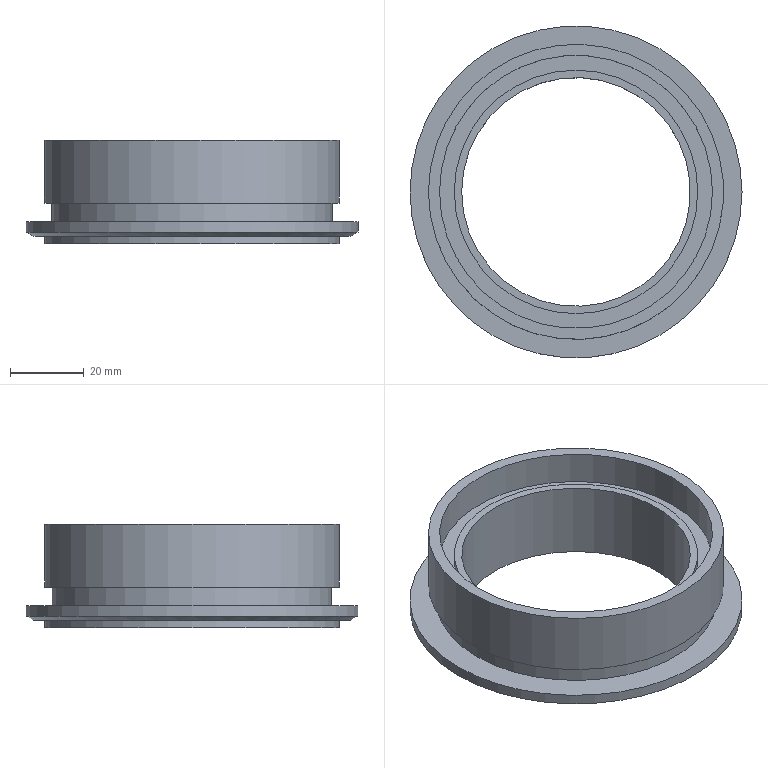Component | NX | CH3404_19_3-2 | 1 solid | 15 faces | box 90 x 90 x 28 mm | volume 48046 mm3 | cylinder 7 | plane 7 | cone 1 | commonest cylinder face diameters 80 x2 90 x1 62 x1 66 x1 74 x1 76 x1
STEP:
#1=CARTESIAN_POINT('',(0.,0.,0.));
#2=DIRECTION('',(0.,0.,1.));
#3=DIRECTION('',(1.,0.,0.));
#4=AXIS2_PLACEMENT_3D('',#1,#2,#3);
#5=CARTESIAN_POINT('',(45.,0.,77.155));
#6=VERTEX_POINT('',#5);
#7=CARTESIAN_POINT('',(-45.,0.,77.155));
#8=VERTEX_POINT('',#7);
#9=CARTESIAN_POINT('',(0.,0.,77.155));
#10=DIRECTION('',(0.,0.,1.));
#11=DIRECTION('',(1.,0.,0.));
#12=AXIS2_PLACEMENT_3D('',#9,#10,#11);
#13=CIRCLE('',#12,45.);
#14=CARTESIAN_POINT('',(0.,0.,74.));
#15=DIRECTION('',(0.,0.,-1.));
#16=DIRECTION('',(-1.,0.,0.));
#17=AXIS2_PLACEMENT_3D('',#14,#15,#16);
#18=CYLINDRICAL_SURFACE('',#17,45.);
#19=CARTESIAN_POINT('',(3.142,-3.155));
#20=DIRECTION('',(-1.,0.));
#21=VECTOR('',#20,1.);
#22=LINE('',#19,#21);
#23=(GEOMETRIC_REPRESENTATION_CONTEXT(2)PARAMETRIC_REPRESENTATION_CONTEXT()REPRESENTATION_CONTEXT('',''));
#24=DEFINITIONAL_REPRESENTATION('',(#22),#23);
#25=PCURVE('',#18,#24);
#26=CARTESIAN_POINT('',(0.,0.,76.));
#27=DIRECTION('',(0.,0.,1.));
#28=DIRECTION('',(1.,0.,0.));
#29=AXIS2_PLACEMENT_3D('',#26,#27,#28);
#30=CONICAL_SURFACE('',#29,43.,1.047);
#31=CARTESIAN_POINT('',(0.,1.155));
#32=DIRECTION('',(1.,0.));
#33=VECTOR('',#32,1.);
#34=LINE('',#31,#33);
#35=(GEOMETRIC_REPRESENTATION_CONTEXT(2)PARAMETRIC_REPRESENTATION_CONTEXT()REPRESENTATION_CONTEXT('',''));
#36=DEFINITIONAL_REPRESENTATION('',(#34),#35);
#37=PCURVE('',#30,#36);
#38=SURFACE_CURVE('',#13,(#25,#37),.PCURVE_S1.);
#39=EDGE_CURVE('',#6,#8,#38,.T.);
#40=ORIENTED_EDGE('',*,*,#39,.T.);
#41=CARTESIAN_POINT('',(-45.,0.,80.));
#42=VERTEX_POINT('',#41);
#43=CARTESIAN_POINT('',(-45.,-0.,80.));
#44=CARTESIAN_POINT('',(-45.,-0.,77.155));
#45=B_SPLINE_CURVE_WITH_KNOTS('',1,(#43,#44),.UNSPECIFIED.,.F.,.F.,(2,2),(-6.,-3.155),.PIECEWISE_BEZIER_KNOTS.);
#46=CARTESIAN_POINT('',(0.,0.));
#47=DIRECTION('',(0.,1.));
#48=VECTOR('',#47,1.);
#49=LINE('',#46,#48);
#50=(GEOMETRIC_REPRESENTATION_CONTEXT(2)PARAMETRIC_REPRESENTATION_CONTEXT()REPRESENTATION_CONTEXT('',''));
#51=DEFINITIONAL_REPRESENTATION('',(#49),#50);
#52=PCURVE('',#18,#51);
#53=CARTESIAN_POINT('',(6.283,0.));
#54=DIRECTION('',(0.,1.));
#55=VECTOR('',#54,1.);
#56=LINE('',#53,#55);
#57=(GEOMETRIC_REPRESENTATION_CONTEXT(2)PARAMETRIC_REPRESENTATION_CONTEXT()REPRESENTATION_CONTEXT('',''));
#58=DEFINITIONAL_REPRESENTATION('',(#56),#57);
#59=PCURVE('',#18,#58);
#60=SEAM_CURVE('',#45,(#52,#59),.PCURVE_S1.);
#61=EDGE_CURVE('',#42,#8,#60,.T.);
#62=ORIENTED_EDGE('',*,*,#61,.F.);
#63=CARTESIAN_POINT('',(0.,0.,80.));
#64=DIRECTION('',(0.,0.,-1.));
#65=DIRECTION('',(-1.,0.,0.));
#66=AXIS2_PLACEMENT_3D('',#63,#64,#65);
#67=CIRCLE('',#66,45.);
#68=CARTESIAN_POINT('',(0.,-6.));
#69=DIRECTION('',(1.,0.));
#70=VECTOR('',#69,1.);
#71=LINE('',#68,#70);
#72=(GEOMETRIC_REPRESENTATION_CONTEXT(2)PARAMETRIC_REPRESENTATION_CONTEXT()REPRESENTATION_CONTEXT('',''));
#73=DEFINITIONAL_REPRESENTATION('',(#71),#72);
#74=PCURVE('',#18,#73);
#75=CARTESIAN_POINT('',(0.,-38.,80.));
#76=DIRECTION('',(0.,0.,-1.));
#77=DIRECTION('',(-1.,0.,0.));
#78=AXIS2_PLACEMENT_3D('',#75,#76,#77);
#79=PLANE('',#78);
#80=CARTESIAN_POINT('',(0.,38.));
#81=DIRECTION('',(1.,0.));
#82=AXIS2_PLACEMENT_2D('',#80,#81);
#83=CIRCLE('',#82,45.);
#84=(GEOMETRIC_REPRESENTATION_CONTEXT(2)PARAMETRIC_REPRESENTATION_CONTEXT()REPRESENTATION_CONTEXT('',''));
#85=DEFINITIONAL_REPRESENTATION('',(#83),#84);
#86=PCURVE('',#79,#85);
#87=SURFACE_CURVE('',#67,(#74,#86),.PCURVE_S1.);
#88=EDGE_CURVE('',#42,#42,#87,.T.);
#89=ORIENTED_EDGE('',*,*,#88,.T.);
#90=ORIENTED_EDGE('',*,*,#61,.T.);
#91=CARTESIAN_POINT('',(0.,0.,77.155));
#92=DIRECTION('',(0.,0.,1.));
#93=DIRECTION('',(1.,0.,0.));
#94=AXIS2_PLACEMENT_3D('',#91,#92,#93);
#95=CIRCLE('',#94,45.);
#96=CARTESIAN_POINT('',(9.425,-3.155));
#97=DIRECTION('',(-1.,0.));
#98=VECTOR('',#97,1.);
#99=LINE('',#96,#98);
#100=(GEOMETRIC_REPRESENTATION_CONTEXT(2)PARAMETRIC_REPRESENTATION_CONTEXT()REPRESENTATION_CONTEXT('',''));
#101=DEFINITIONAL_REPRESENTATION('',(#99),#100);
#102=PCURVE('',#18,#101);
#103=CARTESIAN_POINT('',(0.,1.155));
#104=DIRECTION('',(1.,0.));
#105=VECTOR('',#104,1.);
#106=LINE('',#103,#105);
#107=(GEOMETRIC_REPRESENTATION_CONTEXT(2)PARAMETRIC_REPRESENTATION_CONTEXT()REPRESENTATION_CONTEXT('',''));
#108=DEFINITIONAL_REPRESENTATION('',(#106),#107);
#109=PCURVE('',#30,#108);
#110=SURFACE_CURVE('',#95,(#102,#109),.PCURVE_S1.);
#111=EDGE_CURVE('',#8,#6,#110,.T.);
#112=ORIENTED_EDGE('',*,*,#111,.T.);
#113=EDGE_LOOP('',(#40,#62,#89,#90,#112));
#114=FACE_BOUND('',#113,.T.);
#115=ADVANCED_FACE('',(#114),#18,.T.);
#116=CARTESIAN_POINT('',(43.,0.,76.));
#117=VERTEX_POINT('',#116);
#118=CARTESIAN_POINT('',(0.,0.,76.));
#119=DIRECTION('',(0.,0.,-1.));
#120=DIRECTION('',(1.,0.,0.));
#121=AXIS2_PLACEMENT_3D('',#118,#119,#120);
#122=CIRCLE('',#121,43.);
#123=CARTESIAN_POINT('',(0.,-45.,76.));
#124=DIRECTION('',(0.,0.,1.));
#125=DIRECTION('',(1.,0.,0.));
#126=AXIS2_PLACEMENT_3D('',#123,#124,#125);
#127=PLANE('',#126);
#128=CARTESIAN_POINT('',(43.,45.));
#129=CARTESIAN_POINT('',(43.,-29.478));
#130=CARTESIAN_POINT('',(-21.5,7.761));
#131=CARTESIAN_POINT('',(-86.,45.));
#132=CARTESIAN_POINT('',(-21.5,82.239));
#133=CARTESIAN_POINT('',(43.,119.478));
#134=CARTESIAN_POINT('',(43.,45.));
#135=(BOUNDED_CURVE()B_SPLINE_CURVE(2,(#128,#129,#130,#131,#132,#133,#134),.UNSPECIFIED.,.T.,.F.)B_SPLINE_CURVE_WITH_KNOTS((1,2,2,2,2,1),(-2.094,0.,2.094,4.189,6.283,8.378),.UNSPECIFIED.)CURVE()GEOMETRIC_REPRESENTATION_ITEM()RATIONAL_B_SPLINE_CURVE((1.,0.5,1.,0.5,1.,0.5,1.))REPRESENTATION_ITEM(''));
#136=(GEOMETRIC_REPRESENTATION_CONTEXT(2)PARAMETRIC_REPRESENTATION_CONTEXT()REPRESENTATION_CONTEXT('',''));
#137=DEFINITIONAL_REPRESENTATION('',(#135),#136);
#138=PCURVE('',#127,#137);
#139=CARTESIAN_POINT('',(6.283,0.));
#140=DIRECTION('',(-1.,0.));
#141=VECTOR('',#140,1.);
#142=LINE('',#139,#141);
#143=(GEOMETRIC_REPRESENTATION_CONTEXT(2)PARAMETRIC_REPRESENTATION_CONTEXT()REPRESENTATION_CONTEXT('',''));
#144=DEFINITIONAL_REPRESENTATION('',(#142),#143);
#145=PCURVE('',#30,#144);
#146=SURFACE_CURVE('',#122,(#138,#145),.PCURVE_S1.);
#147=EDGE_CURVE('',#117,#117,#146,.T.);
#148=ORIENTED_EDGE('',*,*,#147,.T.);
#149=EDGE_LOOP('',(#148));
#150=FACE_BOUND('',#149,.T.);
#151=CARTESIAN_POINT('',(-40.,0.,76.));
#152=VERTEX_POINT('',#151);
#153=CARTESIAN_POINT('',(0.,0.,76.));
#154=DIRECTION('',(0.,0.,-1.));
#155=DIRECTION('',(-1.,0.,0.));
#156=AXIS2_PLACEMENT_3D('',#153,#154,#155);
#157=CIRCLE('',#156,40.);
#158=CARTESIAN_POINT('',(-40.,45.));
#159=CARTESIAN_POINT('',(-40.,114.282));
#160=CARTESIAN_POINT('',(20.,79.641));
#161=CARTESIAN_POINT('',(80.,45.));
#162=CARTESIAN_POINT('',(20.,10.359));
#163=CARTESIAN_POINT('',(-40.,-24.282));
#164=CARTESIAN_POINT('',(-40.,45.));
#165=(BOUNDED_CURVE()B_SPLINE_CURVE(2,(#158,#159,#160,#161,#162,#163,#164),.UNSPECIFIED.,.T.,.F.)B_SPLINE_CURVE_WITH_KNOTS((1,2,2,2,2,1),(-2.094,0.,2.094,4.189,6.283,8.378),.UNSPECIFIED.)CURVE()GEOMETRIC_REPRESENTATION_ITEM()RATIONAL_B_SPLINE_CURVE((1.,0.5,1.,0.5,1.,0.5,1.))REPRESENTATION_ITEM(''));
#166=(GEOMETRIC_REPRESENTATION_CONTEXT(2)PARAMETRIC_REPRESENTATION_CONTEXT()REPRESENTATION_CONTEXT('',''));
#167=DEFINITIONAL_REPRESENTATION('',(#165),#166);
#168=PCURVE('',#127,#167);
#169=CARTESIAN_POINT('',(0.,0.,74.));
#170=DIRECTION('',(0.,0.,-1.));
#171=DIRECTION('',(-1.,0.,0.));
#172=AXIS2_PLACEMENT_3D('',#169,#170,#171);
#173=CYLINDRICAL_SURFACE('',#172,40.);
#174=CARTESIAN_POINT('',(0.,-2.));
#175=DIRECTION('',(1.,0.));
#176=VECTOR('',#175,1.);
#177=LINE('',#174,#176);
#178=(GEOMETRIC_REPRESENTATION_CONTEXT(2)PARAMETRIC_REPRESENTATION_CONTEXT()REPRESENTATION_CONTEXT('',''));
#179=DEFINITIONAL_REPRESENTATION('',(#177),#178);
#180=PCURVE('',#173,#179);
#181=SURFACE_CURVE('',#157,(#168,#180),.PCURVE_S1.);
#182=EDGE_CURVE('',#152,#152,#181,.T.);
#183=ORIENTED_EDGE('',*,*,#182,.F.);
#184=EDGE_LOOP('',(#183));
#185=FACE_BOUND('',#184,.T.);
#186=ADVANCED_FACE('',(#150,#185),#127,.F.);
#187=CARTESIAN_POINT('',(-40.,0.,74.));
#188=VERTEX_POINT('',#187);
#189=CARTESIAN_POINT('',(0.,0.,74.));
#190=DIRECTION('',(0.,0.,-1.));
#191=DIRECTION('',(-1.,0.,0.));
#192=AXIS2_PLACEMENT_3D('',#189,#190,#191);
#193=CIRCLE('',#192,40.);
#194=CARTESIAN_POINT('',(0.,0.));
#195=DIRECTION('',(1.,0.));
#196=VECTOR('',#195,1.);
#197=LINE('',#194,#196);
#198=(GEOMETRIC_REPRESENTATION_CONTEXT(2)PARAMETRIC_REPRESENTATION_CONTEXT()REPRESENTATION_CONTEXT('',''));
#199=DEFINITIONAL_REPRESENTATION('',(#197),#198);
#200=PCURVE('',#173,#199);
#201=CARTESIAN_POINT('',(0.,-40.,74.));
#202=DIRECTION('',(0.,0.,1.));
#203=DIRECTION('',(1.,0.,0.));
#204=AXIS2_PLACEMENT_3D('',#201,#202,#203);
#205=PLANE('',#204);
#206=CARTESIAN_POINT('',(-40.,40.));
#207=CARTESIAN_POINT('',(-40.,109.282));
#208=CARTESIAN_POINT('',(20.,74.641));
#209=CARTESIAN_POINT('',(80.,40.));
#210=CARTESIAN_POINT('',(20.,5.359));
#211=CARTESIAN_POINT('',(-40.,-29.282));
#212=CARTESIAN_POINT('',(-40.,40.));
#213=(BOUNDED_CURVE()B_SPLINE_CURVE(2,(#206,#207,#208,#209,#210,#211,#212),.UNSPECIFIED.,.T.,.F.)B_SPLINE_CURVE_WITH_KNOTS((1,2,2,2,2,1),(-2.094,0.,2.094,4.189,6.283,8.378),.UNSPECIFIED.)CURVE()GEOMETRIC_REPRESENTATION_ITEM()RATIONAL_B_SPLINE_CURVE((1.,0.5,1.,0.5,1.,0.5,1.))REPRESENTATION_ITEM(''));
#214=(GEOMETRIC_REPRESENTATION_CONTEXT(2)PARAMETRIC_REPRESENTATION_CONTEXT()REPRESENTATION_CONTEXT('',''));
#215=DEFINITIONAL_REPRESENTATION('',(#213),#214);
#216=PCURVE('',#205,#215);
#217=SURFACE_CURVE('',#193,(#200,#216),.PCURVE_S1.);
#218=EDGE_CURVE('',#188,#188,#217,.T.);
#219=ORIENTED_EDGE('',*,*,#218,.F.);
#220=CARTESIAN_POINT('',(-40.,-0.,76.));
#221=CARTESIAN_POINT('',(-40.,-0.,74.));
#222=B_SPLINE_CURVE_WITH_KNOTS('',1,(#220,#221),.UNSPECIFIED.,.F.,.F.,(2,2),(-2.,0.),.PIECEWISE_BEZIER_KNOTS.);
#223=CARTESIAN_POINT('',(0.,0.));
#224=DIRECTION('',(0.,1.));
#225=VECTOR('',#224,1.);
#226=LINE('',#223,#225);
#227=(GEOMETRIC_REPRESENTATION_CONTEXT(2)PARAMETRIC_REPRESENTATION_CONTEXT()REPRESENTATION_CONTEXT('',''));
#228=DEFINITIONAL_REPRESENTATION('',(#226),#227);
#229=PCURVE('',#173,#228);
#230=CARTESIAN_POINT('',(6.283,0.));
#231=DIRECTION('',(0.,1.));
#232=VECTOR('',#231,1.);
#233=LINE('',#230,#232);
#234=(GEOMETRIC_REPRESENTATION_CONTEXT(2)PARAMETRIC_REPRESENTATION_CONTEXT()REPRESENTATION_CONTEXT('',''));
#235=DEFINITIONAL_REPRESENTATION('',(#233),#234);
#236=PCURVE('',#173,#235);
#237=SEAM_CURVE('',#222,(#229,#236),.PCURVE_S1.);
#238=EDGE_CURVE('',#152,#188,#237,.T.);
#239=ORIENTED_EDGE('',*,*,#238,.F.);
#240=ORIENTED_EDGE('',*,*,#182,.T.);
#241=ORIENTED_EDGE('',*,*,#238,.T.);
#242=EDGE_LOOP('',(#219,#239,#240,#241));
#243=FACE_BOUND('',#242,.T.);
#244=ADVANCED_FACE('',(#243),#173,.T.);
#245=CARTESIAN_POINT('',(-31.,0.,74.));
#246=VERTEX_POINT('',#245);
#247=CARTESIAN_POINT('',(0.,0.,74.));
#248=DIRECTION('',(0.,0.,-1.));
#249=DIRECTION('',(-1.,0.,0.));
#250=AXIS2_PLACEMENT_3D('',#247,#248,#249);
#251=CIRCLE('',#250,31.);
#252=CARTESIAN_POINT('',(-31.,40.));
#253=CARTESIAN_POINT('',(-31.,93.694));
#254=CARTESIAN_POINT('',(15.5,66.847));
#255=CARTESIAN_POINT('',(62.,40.));
#256=CARTESIAN_POINT('',(15.5,13.153));
#257=CARTESIAN_POINT('',(-31.,-13.694));
#258=CARTESIAN_POINT('',(-31.,40.));
#259=(BOUNDED_CURVE()B_SPLINE_CURVE(2,(#252,#253,#254,#255,#256,#257,#258),.UNSPECIFIED.,.T.,.F.)B_SPLINE_CURVE_WITH_KNOTS((1,2,2,2,2,1),(-2.094,0.,2.094,4.189,6.283,8.378),.UNSPECIFIED.)CURVE()GEOMETRIC_REPRESENTATION_ITEM()RATIONAL_B_SPLINE_CURVE((1.,0.5,1.,0.5,1.,0.5,1.))REPRESENTATION_ITEM(''));
#260=(GEOMETRIC_REPRESENTATION_CONTEXT(2)PARAMETRIC_REPRESENTATION_CONTEXT()REPRESENTATION_CONTEXT('',''));
#261=DEFINITIONAL_REPRESENTATION('',(#259),#260);
#262=PCURVE('',#205,#261);
#263=CARTESIAN_POINT('',(0.,0.,74.));
#264=DIRECTION('',(0.,0.,-1.));
#265=DIRECTION('',(-1.,0.,0.));
#266=AXIS2_PLACEMENT_3D('',#263,#264,#265);
#267=CYLINDRICAL_SURFACE('',#266,31.);
#268=CARTESIAN_POINT('',(0.,0.));
#269=DIRECTION('',(1.,0.));
#270=VECTOR('',#269,1.);
#271=LINE('',#268,#270);
#272=(GEOMETRIC_REPRESENTATION_CONTEXT(2)PARAMETRIC_REPRESENTATION_CONTEXT()REPRESENTATION_CONTEXT('',''));
#273=DEFINITIONAL_REPRESENTATION('',(#271),#272);
#274=PCURVE('',#267,#273);
#275=SURFACE_CURVE('',#251,(#262,#274),.PCURVE_S1.);
#276=EDGE_CURVE('',#246,#246,#275,.T.);
#277=ORIENTED_EDGE('',*,*,#276,.F.);
#278=EDGE_LOOP('',(#277));
#279=FACE_BOUND('',#278,.T.);
#280=ORIENTED_EDGE('',*,*,#218,.T.);
#281=EDGE_LOOP('',(#280));
#282=FACE_BOUND('',#281,.T.);
#283=ADVANCED_FACE('',(#279,#282),#205,.F.);
#284=CARTESIAN_POINT('',(-31.,0.,95.));
#285=VERTEX_POINT('',#284);
#286=CARTESIAN_POINT('',(0.,0.,95.));
#287=DIRECTION('',(0.,0.,-1.));
#288=DIRECTION('',(-1.,0.,0.));
#289=AXIS2_PLACEMENT_3D('',#286,#287,#288);
#290=CIRCLE('',#289,31.);
#291=CARTESIAN_POINT('',(0.,-21.));
#292=DIRECTION('',(1.,0.));
#293=VECTOR('',#292,1.);
#294=LINE('',#291,#293);
#295=(GEOMETRIC_REPRESENTATION_CONTEXT(2)PARAMETRIC_REPRESENTATION_CONTEXT()REPRESENTATION_CONTEXT('',''));
#296=DEFINITIONAL_REPRESENTATION('',(#294),#295);
#297=PCURVE('',#267,#296);
#298=CARTESIAN_POINT('',(0.,-31.,95.));
#299=DIRECTION('',(0.,0.,-1.));
#300=DIRECTION('',(-1.,0.,0.));
#301=AXIS2_PLACEMENT_3D('',#298,#299,#300);
#302=PLANE('',#301);
#303=CARTESIAN_POINT('',(0.,31.));
#304=DIRECTION('',(1.,0.));
#305=AXIS2_PLACEMENT_2D('',#303,#304);
#306=CIRCLE('',#305,31.);
#307=(GEOMETRIC_REPRESENTATION_CONTEXT(2)PARAMETRIC_REPRESENTATION_CONTEXT()REPRESENTATION_CONTEXT('',''));
#308=DEFINITIONAL_REPRESENTATION('',(#306),#307);
#309=PCURVE('',#302,#308);
#310=SURFACE_CURVE('',#290,(#297,#309),.PCURVE_S1.);
#311=EDGE_CURVE('',#285,#285,#310,.T.);
#312=ORIENTED_EDGE('',*,*,#311,.T.);
#313=CARTESIAN_POINT('',(-31.,0.,95.));
#314=CARTESIAN_POINT('',(-31.,0.,74.));
#315=B_SPLINE_CURVE_WITH_KNOTS('',1,(#313,#314),.UNSPECIFIED.,.F.,.F.,(2,2),(-21.,0.),.PIECEWISE_BEZIER_KNOTS.);
#316=CARTESIAN_POINT('',(6.283,0.));
#317=DIRECTION('',(0.,1.));
#318=VECTOR('',#317,1.);
#319=LINE('',#316,#318);
#320=(GEOMETRIC_REPRESENTATION_CONTEXT(2)PARAMETRIC_REPRESENTATION_CONTEXT()REPRESENTATION_CONTEXT('',''));
#321=DEFINITIONAL_REPRESENTATION('',(#319),#320);
#322=PCURVE('',#267,#321);
#323=CARTESIAN_POINT('',(0.,0.));
#324=DIRECTION('',(0.,1.));
#325=VECTOR('',#324,1.);
#326=LINE('',#323,#325);
#327=(GEOMETRIC_REPRESENTATION_CONTEXT(2)PARAMETRIC_REPRESENTATION_CONTEXT()REPRESENTATION_CONTEXT('',''));
#328=DEFINITIONAL_REPRESENTATION('',(#326),#327);
#329=PCURVE('',#267,#328);
#330=SEAM_CURVE('',#315,(#322,#329),.PCURVE_S1.);
#331=EDGE_CURVE('',#285,#246,#330,.T.);
#332=ORIENTED_EDGE('',*,*,#331,.T.);
#333=ORIENTED_EDGE('',*,*,#276,.F.);
#334=ORIENTED_EDGE('',*,*,#331,.F.);
#335=EDGE_LOOP('',(#312,#332,#333,#334));
#336=FACE_BOUND('',#335,.F.);
#337=ADVANCED_FACE('',(#336),#267,.F.);
#338=CARTESIAN_POINT('',(-33.,0.,95.));
#339=VERTEX_POINT('',#338);
#340=CARTESIAN_POINT('',(0.,0.,95.));
#341=DIRECTION('',(0.,0.,-1.));
#342=DIRECTION('',(-1.,0.,0.));
#343=AXIS2_PLACEMENT_3D('',#340,#341,#342);
#344=CIRCLE('',#343,33.);
#345=CARTESIAN_POINT('',(0.,31.));
#346=DIRECTION('',(1.,0.));
#347=AXIS2_PLACEMENT_2D('',#345,#346);
#348=CIRCLE('',#347,33.);
#349=(GEOMETRIC_REPRESENTATION_CONTEXT(2)PARAMETRIC_REPRESENTATION_CONTEXT()REPRESENTATION_CONTEXT('',''));
#350=DEFINITIONAL_REPRESENTATION('',(#348),#349);
#351=PCURVE('',#302,#350);
#352=CARTESIAN_POINT('',(0.,0.,74.));
#353=DIRECTION('',(0.,0.,-1.));
#354=DIRECTION('',(-1.,0.,0.));
#355=AXIS2_PLACEMENT_3D('',#352,#353,#354);
#356=CYLINDRICAL_SURFACE('',#355,33.);
#357=CARTESIAN_POINT('',(0.,-21.));
#358=DIRECTION('',(1.,0.));
#359=VECTOR('',#358,1.);
#360=LINE('',#357,#359);
#361=(GEOMETRIC_REPRESENTATION_CONTEXT(2)PARAMETRIC_REPRESENTATION_CONTEXT()REPRESENTATION_CONTEXT('',''));
#362=DEFINITIONAL_REPRESENTATION('',(#360),#361);
#363=PCURVE('',#356,#362);
#364=SURFACE_CURVE('',#344,(#351,#363),.PCURVE_S1.);
#365=EDGE_CURVE('',#339,#339,#364,.T.);
#366=ORIENTED_EDGE('',*,*,#365,.F.);
#367=EDGE_LOOP('',(#366));
#368=FACE_BOUND('',#367,.T.);
#369=ORIENTED_EDGE('',*,*,#311,.T.);
#370=EDGE_LOOP('',(#369));
#371=FACE_BOUND('',#370,.T.);
#372=ADVANCED_FACE('',(#368,#371),#302,.F.);
#373=CARTESIAN_POINT('',(-33.,0.,93.));
#374=VERTEX_POINT('',#373);
#375=CARTESIAN_POINT('',(0.,0.,93.));
#376=DIRECTION('',(0.,0.,-1.));
#377=DIRECTION('',(-1.,0.,0.));
#378=AXIS2_PLACEMENT_3D('',#375,#376,#377);
#379=CIRCLE('',#378,33.);
#380=CARTESIAN_POINT('',(0.,-19.));
#381=DIRECTION('',(1.,0.));
#382=VECTOR('',#381,1.);
#383=LINE('',#380,#382);
#384=(GEOMETRIC_REPRESENTATION_CONTEXT(2)PARAMETRIC_REPRESENTATION_CONTEXT()REPRESENTATION_CONTEXT('',''));
#385=DEFINITIONAL_REPRESENTATION('',(#383),#384);
#386=PCURVE('',#356,#385);
#387=CARTESIAN_POINT('',(0.,-33.,93.));
#388=DIRECTION('',(0.,0.,-1.));
#389=DIRECTION('',(-1.,0.,0.));
#390=AXIS2_PLACEMENT_3D('',#387,#388,#389);
#391=PLANE('',#390);
#392=CARTESIAN_POINT('',(0.,33.));
#393=DIRECTION('',(1.,0.));
#394=AXIS2_PLACEMENT_2D('',#392,#393);
#395=CIRCLE('',#394,33.);
#396=(GEOMETRIC_REPRESENTATION_CONTEXT(2)PARAMETRIC_REPRESENTATION_CONTEXT()REPRESENTATION_CONTEXT('',''));
#397=DEFINITIONAL_REPRESENTATION('',(#395),#396);
#398=PCURVE('',#391,#397);
#399=SURFACE_CURVE('',#379,(#386,#398),.PCURVE_S1.);
#400=EDGE_CURVE('',#374,#374,#399,.T.);
#401=ORIENTED_EDGE('',*,*,#400,.F.);
#402=CARTESIAN_POINT('',(-33.,-0.,95.));
#403=CARTESIAN_POINT('',(-33.,-0.,93.));
#404=B_SPLINE_CURVE_WITH_KNOTS('',1,(#402,#403),.UNSPECIFIED.,.F.,.F.,(2,2),(-21.,-19.),.PIECEWISE_BEZIER_KNOTS.);
#405=CARTESIAN_POINT('',(0.,0.));
#406=DIRECTION('',(0.,1.));
#407=VECTOR('',#406,1.);
#408=LINE('',#405,#407);
#409=(GEOMETRIC_REPRESENTATION_CONTEXT(2)PARAMETRIC_REPRESENTATION_CONTEXT()REPRESENTATION_CONTEXT('',''));
#410=DEFINITIONAL_REPRESENTATION('',(#408),#409);
#411=PCURVE('',#356,#410);
#412=CARTESIAN_POINT('',(6.283,0.));
#413=DIRECTION('',(0.,1.));
#414=VECTOR('',#413,1.);
#415=LINE('',#412,#414);
#416=(GEOMETRIC_REPRESENTATION_CONTEXT(2)PARAMETRIC_REPRESENTATION_CONTEXT()REPRESENTATION_CONTEXT('',''));
#417=DEFINITIONAL_REPRESENTATION('',(#415),#416);
#418=PCURVE('',#356,#417);
#419=SEAM_CURVE('',#404,(#411,#418),.PCURVE_S1.);
#420=EDGE_CURVE('',#339,#374,#419,.T.);
#421=ORIENTED_EDGE('',*,*,#420,.F.);
#422=ORIENTED_EDGE('',*,*,#365,.T.);
#423=ORIENTED_EDGE('',*,*,#420,.T.);
#424=EDGE_LOOP('',(#401,#421,#422,#423));
#425=FACE_BOUND('',#424,.T.);
#426=ADVANCED_FACE('',(#425),#356,.T.);
#427=CARTESIAN_POINT('',(-37.,0.,93.));
#428=VERTEX_POINT('',#427);
#429=CARTESIAN_POINT('',(0.,0.,93.));
#430=DIRECTION('',(0.,0.,-1.));
#431=DIRECTION('',(-1.,0.,0.));
#432=AXIS2_PLACEMENT_3D('',#429,#430,#431);
#433=CIRCLE('',#432,37.);
#434=CARTESIAN_POINT('',(0.,33.));
#435=DIRECTION('',(1.,0.));
#436=AXIS2_PLACEMENT_2D('',#434,#435);
#437=CIRCLE('',#436,37.);
#438=(GEOMETRIC_REPRESENTATION_CONTEXT(2)PARAMETRIC_REPRESENTATION_CONTEXT()REPRESENTATION_CONTEXT('',''));
#439=DEFINITIONAL_REPRESENTATION('',(#437),#438);
#440=PCURVE('',#391,#439);
#441=CARTESIAN_POINT('',(0.,0.,74.));
#442=DIRECTION('',(0.,0.,-1.));
#443=DIRECTION('',(-1.,0.,0.));
#444=AXIS2_PLACEMENT_3D('',#441,#442,#443);
#445=CYLINDRICAL_SURFACE('',#444,37.);
#446=CARTESIAN_POINT('',(0.,-19.));
#447=DIRECTION('',(1.,0.));
#448=VECTOR('',#447,1.);
#449=LINE('',#446,#448);
#450=(GEOMETRIC_REPRESENTATION_CONTEXT(2)PARAMETRIC_REPRESENTATION_CONTEXT()REPRESENTATION_CONTEXT('',''));
#451=DEFINITIONAL_REPRESENTATION('',(#449),#450);
#452=PCURVE('',#445,#451);
#453=SURFACE_CURVE('',#433,(#440,#452),.PCURVE_S1.);
#454=EDGE_CURVE('',#428,#428,#453,.T.);
#455=ORIENTED_EDGE('',*,*,#454,.F.);
#456=EDGE_LOOP('',(#455));
#457=FACE_BOUND('',#456,.T.);
#458=ORIENTED_EDGE('',*,*,#400,.T.);
#459=EDGE_LOOP('',(#458));
#460=FACE_BOUND('',#459,.T.);
#461=ADVANCED_FACE('',(#457,#460),#391,.F.);
#462=CARTESIAN_POINT('',(-37.,0.,102.));
#463=VERTEX_POINT('',#462);
#464=CARTESIAN_POINT('',(0.,0.,102.));
#465=DIRECTION('',(0.,0.,-1.));
#466=DIRECTION('',(-1.,0.,0.));
#467=AXIS2_PLACEMENT_3D('',#464,#465,#466);
#468=CIRCLE('',#467,37.);
#469=CARTESIAN_POINT('',(0.,-28.));
#470=DIRECTION('',(1.,0.));
#471=VECTOR('',#470,1.);
#472=LINE('',#469,#471);
#473=(GEOMETRIC_REPRESENTATION_CONTEXT(2)PARAMETRIC_REPRESENTATION_CONTEXT()REPRESENTATION_CONTEXT('',''));
#474=DEFINITIONAL_REPRESENTATION('',(#472),#473);
#475=PCURVE('',#445,#474);
#476=CARTESIAN_POINT('',(0.,-37.,102.));
#477=DIRECTION('',(0.,0.,-1.));
#478=DIRECTION('',(-1.,0.,0.));
#479=AXIS2_PLACEMENT_3D('',#476,#477,#478);
#480=PLANE('',#479);
#481=CARTESIAN_POINT('',(0.,37.));
#482=DIRECTION('',(1.,0.));
#483=AXIS2_PLACEMENT_2D('',#481,#482);
#484=CIRCLE('',#483,37.);
#485=(GEOMETRIC_REPRESENTATION_CONTEXT(2)PARAMETRIC_REPRESENTATION_CONTEXT()REPRESENTATION_CONTEXT('',''));
#486=DEFINITIONAL_REPRESENTATION('',(#484),#485);
#487=PCURVE('',#480,#486);
#488=SURFACE_CURVE('',#468,(#475,#487),.PCURVE_S1.);
#489=EDGE_CURVE('',#463,#463,#488,.T.);
#490=ORIENTED_EDGE('',*,*,#489,.T.);
#491=CARTESIAN_POINT('',(-37.,0.,102.));
#492=CARTESIAN_POINT('',(-37.,0.,93.));
#493=B_SPLINE_CURVE_WITH_KNOTS('',1,(#491,#492),.UNSPECIFIED.,.F.,.F.,(2,2),(-28.,-19.),.PIECEWISE_BEZIER_KNOTS.);
#494=CARTESIAN_POINT('',(6.283,0.));
#495=DIRECTION('',(0.,1.));
#496=VECTOR('',#495,1.);
#497=LINE('',#494,#496);
#498=(GEOMETRIC_REPRESENTATION_CONTEXT(2)PARAMETRIC_REPRESENTATION_CONTEXT()REPRESENTATION_CONTEXT('',''));
#499=DEFINITIONAL_REPRESENTATION('',(#497),#498);
#500=PCURVE('',#445,#499);
#501=CARTESIAN_POINT('',(0.,0.));
#502=DIRECTION('',(0.,1.));
#503=VECTOR('',#502,1.);
#504=LINE('',#501,#503);
#505=(GEOMETRIC_REPRESENTATION_CONTEXT(2)PARAMETRIC_REPRESENTATION_CONTEXT()REPRESENTATION_CONTEXT('',''));
#506=DEFINITIONAL_REPRESENTATION('',(#504),#505);
#507=PCURVE('',#445,#506);
#508=SEAM_CURVE('',#493,(#500,#507),.PCURVE_S1.);
#509=EDGE_CURVE('',#463,#428,#508,.T.);
#510=ORIENTED_EDGE('',*,*,#509,.T.);
#511=ORIENTED_EDGE('',*,*,#454,.F.);
#512=ORIENTED_EDGE('',*,*,#509,.F.);
#513=EDGE_LOOP('',(#490,#510,#511,#512));
#514=FACE_BOUND('',#513,.F.);
#515=ADVANCED_FACE('',(#514),#445,.F.);
#516=CARTESIAN_POINT('',(-40.,0.,102.));
#517=VERTEX_POINT('',#516);
#518=CARTESIAN_POINT('',(0.,0.,102.));
#519=DIRECTION('',(0.,0.,-1.));
#520=DIRECTION('',(-1.,0.,0.));
#521=AXIS2_PLACEMENT_3D('',#518,#519,#520);
#522=CIRCLE('',#521,40.);
#523=CARTESIAN_POINT('',(0.,37.));
#524=DIRECTION('',(1.,0.));
#525=AXIS2_PLACEMENT_2D('',#523,#524);
#526=CIRCLE('',#525,40.);
#527=(GEOMETRIC_REPRESENTATION_CONTEXT(2)PARAMETRIC_REPRESENTATION_CONTEXT()REPRESENTATION_CONTEXT('',''));
#528=DEFINITIONAL_REPRESENTATION('',(#526),#527);
#529=PCURVE('',#480,#528);
#530=CARTESIAN_POINT('',(0.,0.,74.));
#531=DIRECTION('',(0.,0.,-1.));
#532=DIRECTION('',(-1.,0.,0.));
#533=AXIS2_PLACEMENT_3D('',#530,#531,#532);
#534=CYLINDRICAL_SURFACE('',#533,40.);
#535=CARTESIAN_POINT('',(0.,-28.));
#536=DIRECTION('',(1.,0.));
#537=VECTOR('',#536,1.);
#538=LINE('',#535,#537);
#539=(GEOMETRIC_REPRESENTATION_CONTEXT(2)PARAMETRIC_REPRESENTATION_CONTEXT()REPRESENTATION_CONTEXT('',''));
#540=DEFINITIONAL_REPRESENTATION('',(#538),#539);
#541=PCURVE('',#534,#540);
#542=SURFACE_CURVE('',#522,(#529,#541),.PCURVE_S1.);
#543=EDGE_CURVE('',#517,#517,#542,.T.);
#544=ORIENTED_EDGE('',*,*,#543,.F.);
#545=EDGE_LOOP('',(#544));
#546=FACE_BOUND('',#545,.T.);
#547=ORIENTED_EDGE('',*,*,#489,.T.);
#548=EDGE_LOOP('',(#547));
#549=FACE_BOUND('',#548,.T.);
#550=ADVANCED_FACE('',(#546,#549),#480,.F.);
#551=CARTESIAN_POINT('',(-40.,0.,85.));
#552=VERTEX_POINT('',#551);
#553=CARTESIAN_POINT('',(0.,0.,85.));
#554=DIRECTION('',(0.,0.,-1.));
#555=DIRECTION('',(-1.,0.,0.));
#556=AXIS2_PLACEMENT_3D('',#553,#554,#555);
#557=CIRCLE('',#556,40.);
#558=CARTESIAN_POINT('',(0.,-11.));
#559=DIRECTION('',(1.,0.));
#560=VECTOR('',#559,1.);
#561=LINE('',#558,#560);
#562=(GEOMETRIC_REPRESENTATION_CONTEXT(2)PARAMETRIC_REPRESENTATION_CONTEXT()REPRESENTATION_CONTEXT('',''));
#563=DEFINITIONAL_REPRESENTATION('',(#561),#562);
#564=PCURVE('',#534,#563);
#565=CARTESIAN_POINT('',(0.,-40.,85.));
#566=DIRECTION('',(0.,0.,1.));
#567=DIRECTION('',(1.,0.,0.));
#568=AXIS2_PLACEMENT_3D('',#565,#566,#567);
#569=PLANE('',#568);
#570=CARTESIAN_POINT('',(-40.,40.));
#571=CARTESIAN_POINT('',(-40.,109.282));
#572=CARTESIAN_POINT('',(20.,74.641));
#573=CARTESIAN_POINT('',(80.,40.));
#574=CARTESIAN_POINT('',(20.,5.359));
#575=CARTESIAN_POINT('',(-40.,-29.282));
#576=CARTESIAN_POINT('',(-40.,40.));
#577=(BOUNDED_CURVE()B_SPLINE_CURVE(2,(#570,#571,#572,#573,#574,#575,#576),.UNSPECIFIED.,.T.,.F.)B_SPLINE_CURVE_WITH_KNOTS((1,2,2,2,2,1),(-2.094,0.,2.094,4.189,6.283,8.378),.UNSPECIFIED.)CURVE()GEOMETRIC_REPRESENTATION_ITEM()RATIONAL_B_SPLINE_CURVE((1.,0.5,1.,0.5,1.,0.5,1.))REPRESENTATION_ITEM(''));
#578=(GEOMETRIC_REPRESENTATION_CONTEXT(2)PARAMETRIC_REPRESENTATION_CONTEXT()REPRESENTATION_CONTEXT('',''));
#579=DEFINITIONAL_REPRESENTATION('',(#577),#578);
#580=PCURVE('',#569,#579);
#581=SURFACE_CURVE('',#557,(#564,#580),.PCURVE_S1.);
#582=EDGE_CURVE('',#552,#552,#581,.T.);
#583=ORIENTED_EDGE('',*,*,#582,.F.);
#584=CARTESIAN_POINT('',(-40.,-0.,102.));
#585=CARTESIAN_POINT('',(-40.,-0.,85.));
#586=B_SPLINE_CURVE_WITH_KNOTS('',1,(#584,#585),.UNSPECIFIED.,.F.,.F.,(2,2),(-28.,-11.),.PIECEWISE_BEZIER_KNOTS.);
#587=CARTESIAN_POINT('',(0.,0.));
#588=DIRECTION('',(0.,1.));
#589=VECTOR('',#588,1.);
#590=LINE('',#587,#589);
#591=(GEOMETRIC_REPRESENTATION_CONTEXT(2)PARAMETRIC_REPRESENTATION_CONTEXT()REPRESENTATION_CONTEXT('',''));
#592=DEFINITIONAL_REPRESENTATION('',(#590),#591);
#593=PCURVE('',#534,#592);
#594=CARTESIAN_POINT('',(6.283,0.));
#595=DIRECTION('',(0.,1.));
#596=VECTOR('',#595,1.);
#597=LINE('',#594,#596);
#598=(GEOMETRIC_REPRESENTATION_CONTEXT(2)PARAMETRIC_REPRESENTATION_CONTEXT()REPRESENTATION_CONTEXT('',''));
#599=DEFINITIONAL_REPRESENTATION('',(#597),#598);
#600=PCURVE('',#534,#599);
#601=SEAM_CURVE('',#586,(#593,#600),.PCURVE_S1.);
#602=EDGE_CURVE('',#517,#552,#601,.T.);
#603=ORIENTED_EDGE('',*,*,#602,.F.);
#604=ORIENTED_EDGE('',*,*,#543,.T.);
#605=ORIENTED_EDGE('',*,*,#602,.T.);
#606=EDGE_LOOP('',(#583,#603,#604,#605));
#607=FACE_BOUND('',#606,.T.);
#608=ADVANCED_FACE('',(#607),#534,.T.);
#609=CARTESIAN_POINT('',(-38.,0.,85.));
#610=VERTEX_POINT('',#609);
#611=CARTESIAN_POINT('',(0.,0.,85.));
#612=DIRECTION('',(0.,0.,-1.));
#613=DIRECTION('',(-1.,0.,0.));
#614=AXIS2_PLACEMENT_3D('',#611,#612,#613);
#615=CIRCLE('',#614,38.);
#616=CARTESIAN_POINT('',(-38.,40.));
#617=CARTESIAN_POINT('',(-38.,105.818));
#618=CARTESIAN_POINT('',(19.,72.909));
#619=CARTESIAN_POINT('',(76.,40.));
#620=CARTESIAN_POINT('',(19.,7.091));
#621=CARTESIAN_POINT('',(-38.,-25.818));
#622=CARTESIAN_POINT('',(-38.,40.));
#623=(BOUNDED_CURVE()B_SPLINE_CURVE(2,(#616,#617,#618,#619,#620,#621,#622),.UNSPECIFIED.,.T.,.F.)B_SPLINE_CURVE_WITH_KNOTS((1,2,2,2,2,1),(-2.094,0.,2.094,4.189,6.283,8.378),.UNSPECIFIED.)CURVE()GEOMETRIC_REPRESENTATION_ITEM()RATIONAL_B_SPLINE_CURVE((1.,0.5,1.,0.5,1.,0.5,1.))REPRESENTATION_ITEM(''));
#624=(GEOMETRIC_REPRESENTATION_CONTEXT(2)PARAMETRIC_REPRESENTATION_CONTEXT()REPRESENTATION_CONTEXT('',''));
#625=DEFINITIONAL_REPRESENTATION('',(#623),#624);
#626=PCURVE('',#569,#625);
#627=CARTESIAN_POINT('',(0.,0.,74.));
#628=DIRECTION('',(0.,0.,-1.));
#629=DIRECTION('',(-1.,0.,0.));
#630=AXIS2_PLACEMENT_3D('',#627,#628,#629);
#631=CYLINDRICAL_SURFACE('',#630,38.);
#632=CARTESIAN_POINT('',(0.,-11.));
#633=DIRECTION('',(1.,0.));
#634=VECTOR('',#633,1.);
#635=LINE('',#632,#634);
#636=(GEOMETRIC_REPRESENTATION_CONTEXT(2)PARAMETRIC_REPRESENTATION_CONTEXT()REPRESENTATION_CONTEXT('',''));
#637=DEFINITIONAL_REPRESENTATION('',(#635),#636);
#638=PCURVE('',#631,#637);
#639=SURFACE_CURVE('',#615,(#626,#638),.PCURVE_S1.);
#640=EDGE_CURVE('',#610,#610,#639,.T.);
#641=ORIENTED_EDGE('',*,*,#640,.F.);
#642=EDGE_LOOP('',(#641));
#643=FACE_BOUND('',#642,.T.);
#644=ORIENTED_EDGE('',*,*,#582,.T.);
#645=EDGE_LOOP('',(#644));
#646=FACE_BOUND('',#645,.T.);
#647=ADVANCED_FACE('',(#643,#646),#569,.F.);
#648=CARTESIAN_POINT('',(-38.,0.,80.));
#649=VERTEX_POINT('',#648);
#650=CARTESIAN_POINT('',(0.,0.,80.));
#651=DIRECTION('',(0.,0.,-1.));
#652=DIRECTION('',(-1.,0.,0.));
#653=AXIS2_PLACEMENT_3D('',#650,#651,#652);
#654=CIRCLE('',#653,38.);
#655=CARTESIAN_POINT('',(0.,-6.));
#656=DIRECTION('',(1.,0.));
#657=VECTOR('',#656,1.);
#658=LINE('',#655,#657);
#659=(GEOMETRIC_REPRESENTATION_CONTEXT(2)PARAMETRIC_REPRESENTATION_CONTEXT()REPRESENTATION_CONTEXT('',''));
#660=DEFINITIONAL_REPRESENTATION('',(#658),#659);
#661=PCURVE('',#631,#660);
#662=CARTESIAN_POINT('',(0.,38.));
#663=DIRECTION('',(1.,0.));
#664=AXIS2_PLACEMENT_2D('',#662,#663);
#665=CIRCLE('',#664,38.);
#666=(GEOMETRIC_REPRESENTATION_CONTEXT(2)PARAMETRIC_REPRESENTATION_CONTEXT()REPRESENTATION_CONTEXT('',''));
#667=DEFINITIONAL_REPRESENTATION('',(#665),#666);
#668=PCURVE('',#79,#667);
#669=SURFACE_CURVE('',#654,(#661,#668),.PCURVE_S1.);
#670=EDGE_CURVE('',#649,#649,#669,.T.);
#671=ORIENTED_EDGE('',*,*,#670,.F.);
#672=CARTESIAN_POINT('',(-38.,-0.,85.));
#673=CARTESIAN_POINT('',(-38.,-0.,80.));
#674=B_SPLINE_CURVE_WITH_KNOTS('',1,(#672,#673),.UNSPECIFIED.,.F.,.F.,(2,2),(-11.,-6.),.PIECEWISE_BEZIER_KNOTS.);
#675=CARTESIAN_POINT('',(0.,0.));
#676=DIRECTION('',(0.,1.));
#677=VECTOR('',#676,1.);
#678=LINE('',#675,#677);
#679=(GEOMETRIC_REPRESENTATION_CONTEXT(2)PARAMETRIC_REPRESENTATION_CONTEXT()REPRESENTATION_CONTEXT('',''));
#680=DEFINITIONAL_REPRESENTATION('',(#678),#679);
#681=PCURVE('',#631,#680);
#682=CARTESIAN_POINT('',(6.283,0.));
#683=DIRECTION('',(0.,1.));
#684=VECTOR('',#683,1.);
#685=LINE('',#682,#684);
#686=(GEOMETRIC_REPRESENTATION_CONTEXT(2)PARAMETRIC_REPRESENTATION_CONTEXT()REPRESENTATION_CONTEXT('',''));
#687=DEFINITIONAL_REPRESENTATION('',(#685),#686);
#688=PCURVE('',#631,#687);
#689=SEAM_CURVE('',#674,(#681,#688),.PCURVE_S1.);
#690=EDGE_CURVE('',#610,#649,#689,.T.);
#691=ORIENTED_EDGE('',*,*,#690,.F.);
#692=ORIENTED_EDGE('',*,*,#640,.T.);
#693=ORIENTED_EDGE('',*,*,#690,.T.);
#694=EDGE_LOOP('',(#671,#691,#692,#693));
#695=FACE_BOUND('',#694,.T.);
#696=ADVANCED_FACE('',(#695),#631,.T.);
#697=ORIENTED_EDGE('',*,*,#88,.F.);
#698=EDGE_LOOP('',(#697));
#699=FACE_BOUND('',#698,.T.);
#700=ORIENTED_EDGE('',*,*,#670,.T.);
#701=EDGE_LOOP('',(#700));
#702=FACE_BOUND('',#701,.T.);
#703=ADVANCED_FACE('',(#699,#702),#79,.F.);
#704=ORIENTED_EDGE('',*,*,#39,.F.);
#705=CARTESIAN_POINT('',(43.,-0.,76.));
#706=CARTESIAN_POINT('',(45.,-0.,77.155));
#707=B_SPLINE_CURVE_WITH_KNOTS('',1,(#705,#706),.UNSPECIFIED.,.F.,.F.,(2,2),(0.,2.309),.PIECEWISE_BEZIER_KNOTS.);
#708=CARTESIAN_POINT('',(0.,0.));
#709=DIRECTION('',(0.,1.));
#710=VECTOR('',#709,1.);
#711=LINE('',#708,#710);
#712=(GEOMETRIC_REPRESENTATION_CONTEXT(2)PARAMETRIC_REPRESENTATION_CONTEXT()REPRESENTATION_CONTEXT('',''));
#713=DEFINITIONAL_REPRESENTATION('',(#711),#712);
#714=PCURVE('',#30,#713);
#715=CARTESIAN_POINT('',(6.283,0.));
#716=DIRECTION('',(0.,1.));
#717=VECTOR('',#716,1.);
#718=LINE('',#715,#717);
#719=(GEOMETRIC_REPRESENTATION_CONTEXT(2)PARAMETRIC_REPRESENTATION_CONTEXT()REPRESENTATION_CONTEXT('',''));
#720=DEFINITIONAL_REPRESENTATION('',(#718),#719);
#721=PCURVE('',#30,#720);
#722=SEAM_CURVE('',#707,(#714,#721),.PCURVE_S1.);
#723=EDGE_CURVE('',#117,#6,#722,.T.);
#724=ORIENTED_EDGE('',*,*,#723,.F.);
#725=ORIENTED_EDGE('',*,*,#147,.F.);
#726=ORIENTED_EDGE('',*,*,#723,.T.);
#727=ORIENTED_EDGE('',*,*,#111,.F.);
#728=EDGE_LOOP('',(#704,#724,#725,#726,#727));
#729=FACE_BOUND('',#728,.T.);
#730=ADVANCED_FACE('',(#729),#30,.T.);
#731=CLOSED_SHELL('',(#115,#186,#244,#283,#337,#372,#426,#461,#515,#550,#608,#647,#696,#703,#730));
#732=MANIFOLD_SOLID_BREP('',#731);
#733=(LENGTH_UNIT()NAMED_UNIT(*)SI_UNIT(.MILLI.,.METRE.));
#734=UNCERTAINTY_MEASURE_WITH_UNIT(LENGTH_MEASURE(0.00001),#733,'','');
#735=(NAMED_UNIT(*)PLANE_ANGLE_UNIT()SI_UNIT($,.RADIAN.));
#736=(NAMED_UNIT(*)SI_UNIT($,.STERADIAN.)SOLID_ANGLE_UNIT());
#737=(GEOMETRIC_REPRESENTATION_CONTEXT(3)GLOBAL_UNCERTAINTY_ASSIGNED_CONTEXT((#734))GLOBAL_UNIT_ASSIGNED_CONTEXT((#733,#735,#736))REPRESENTATION_CONTEXT('',''));
#738=ADVANCED_BREP_SHAPE_REPRESENTATION('',(#4,#732),#737);